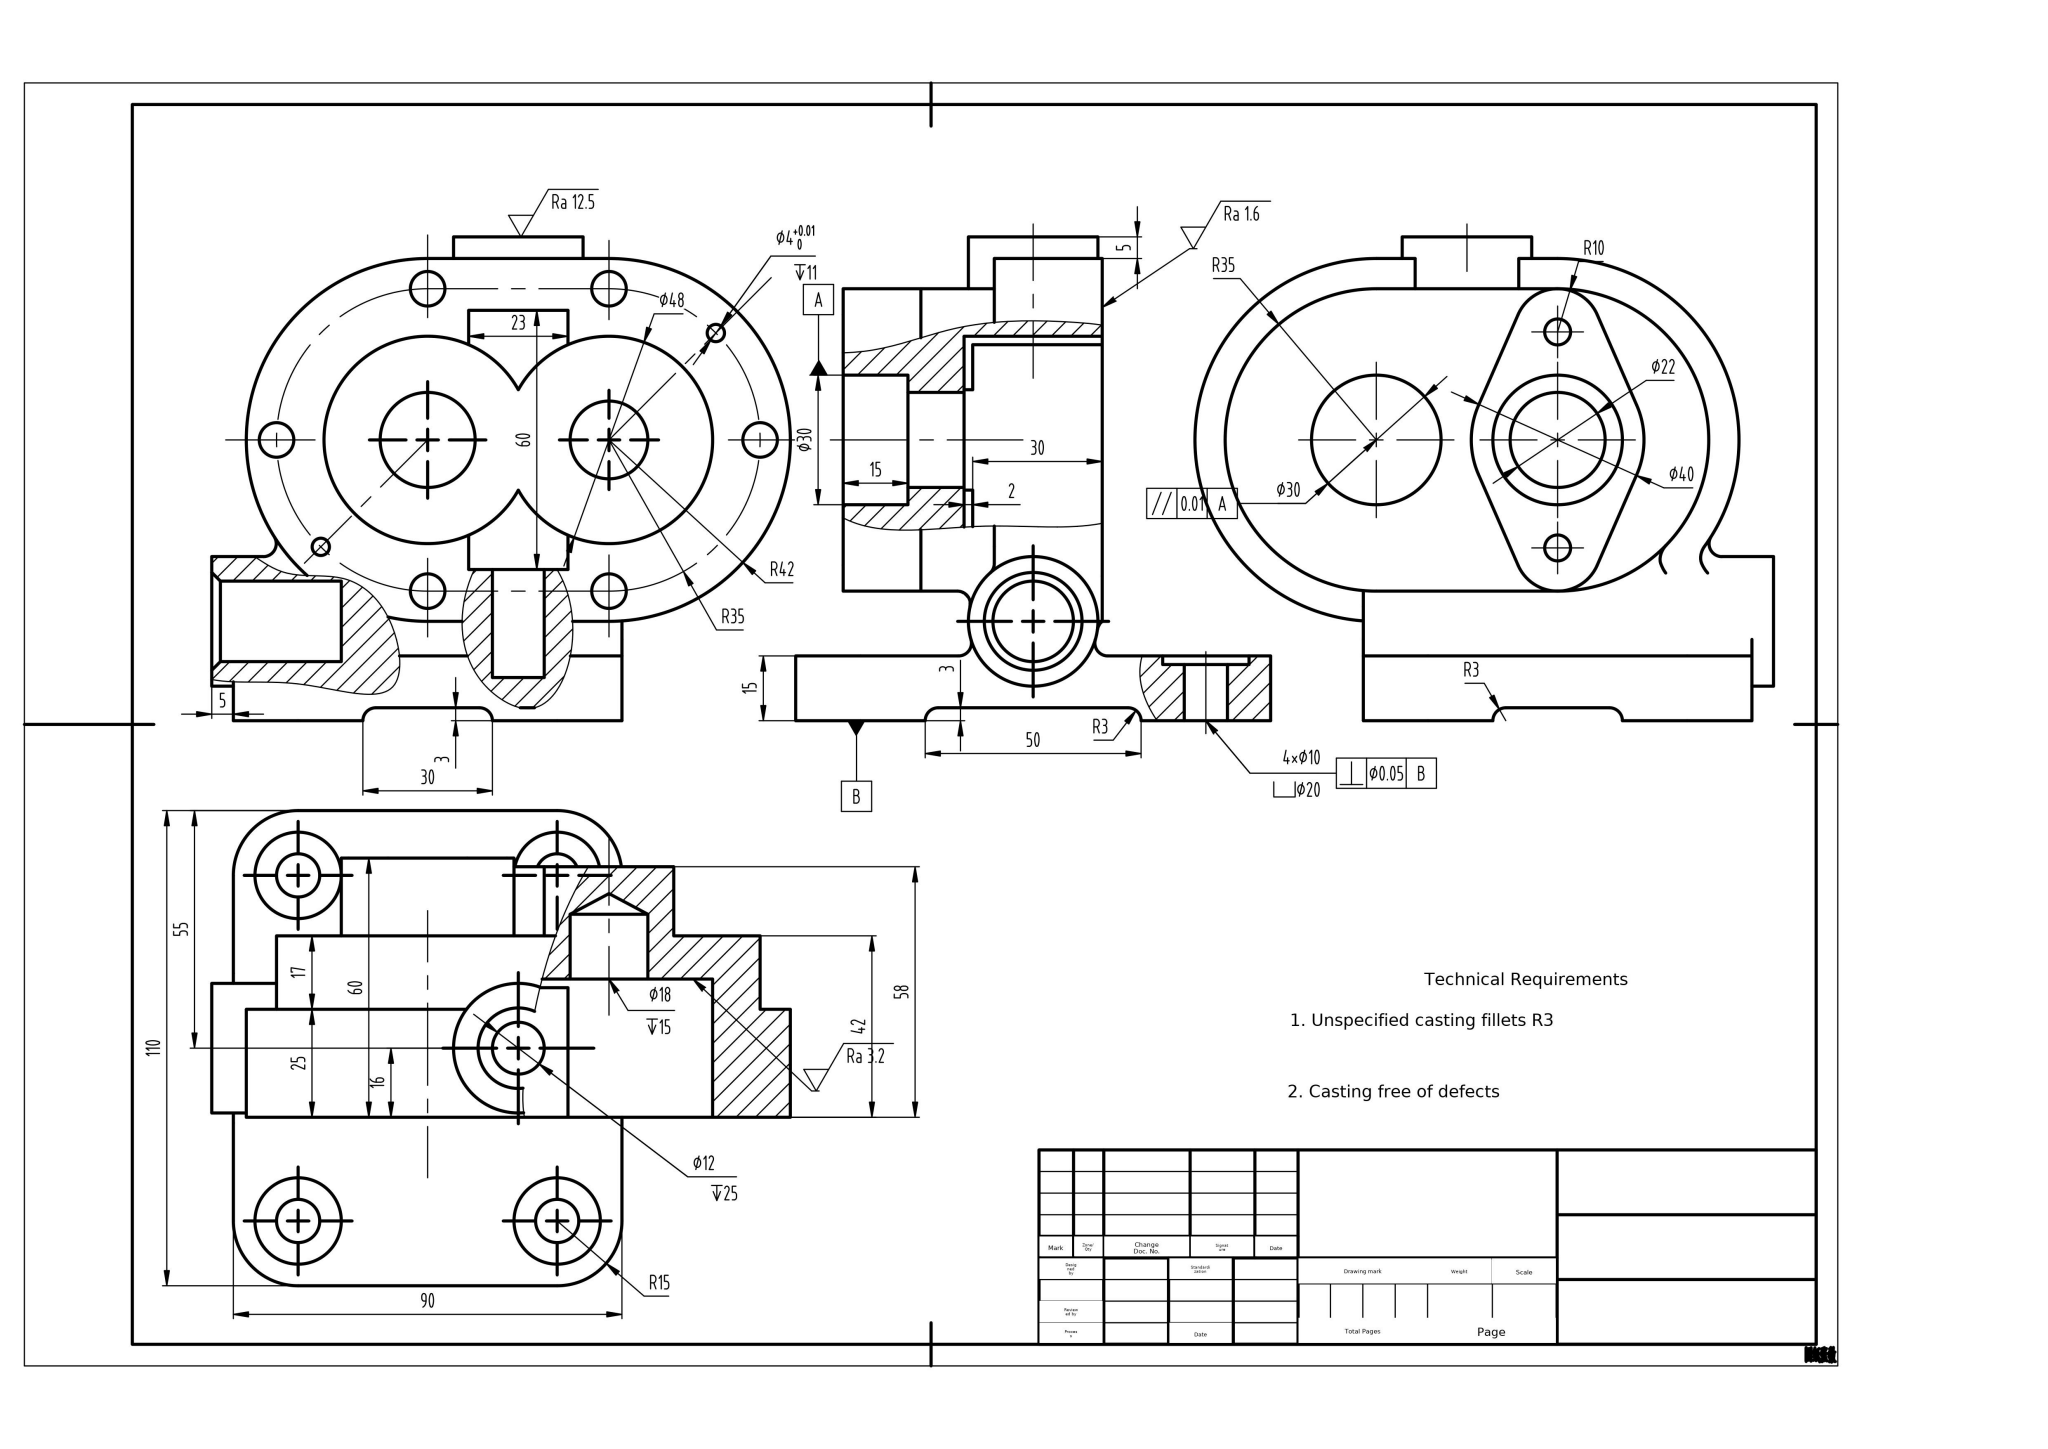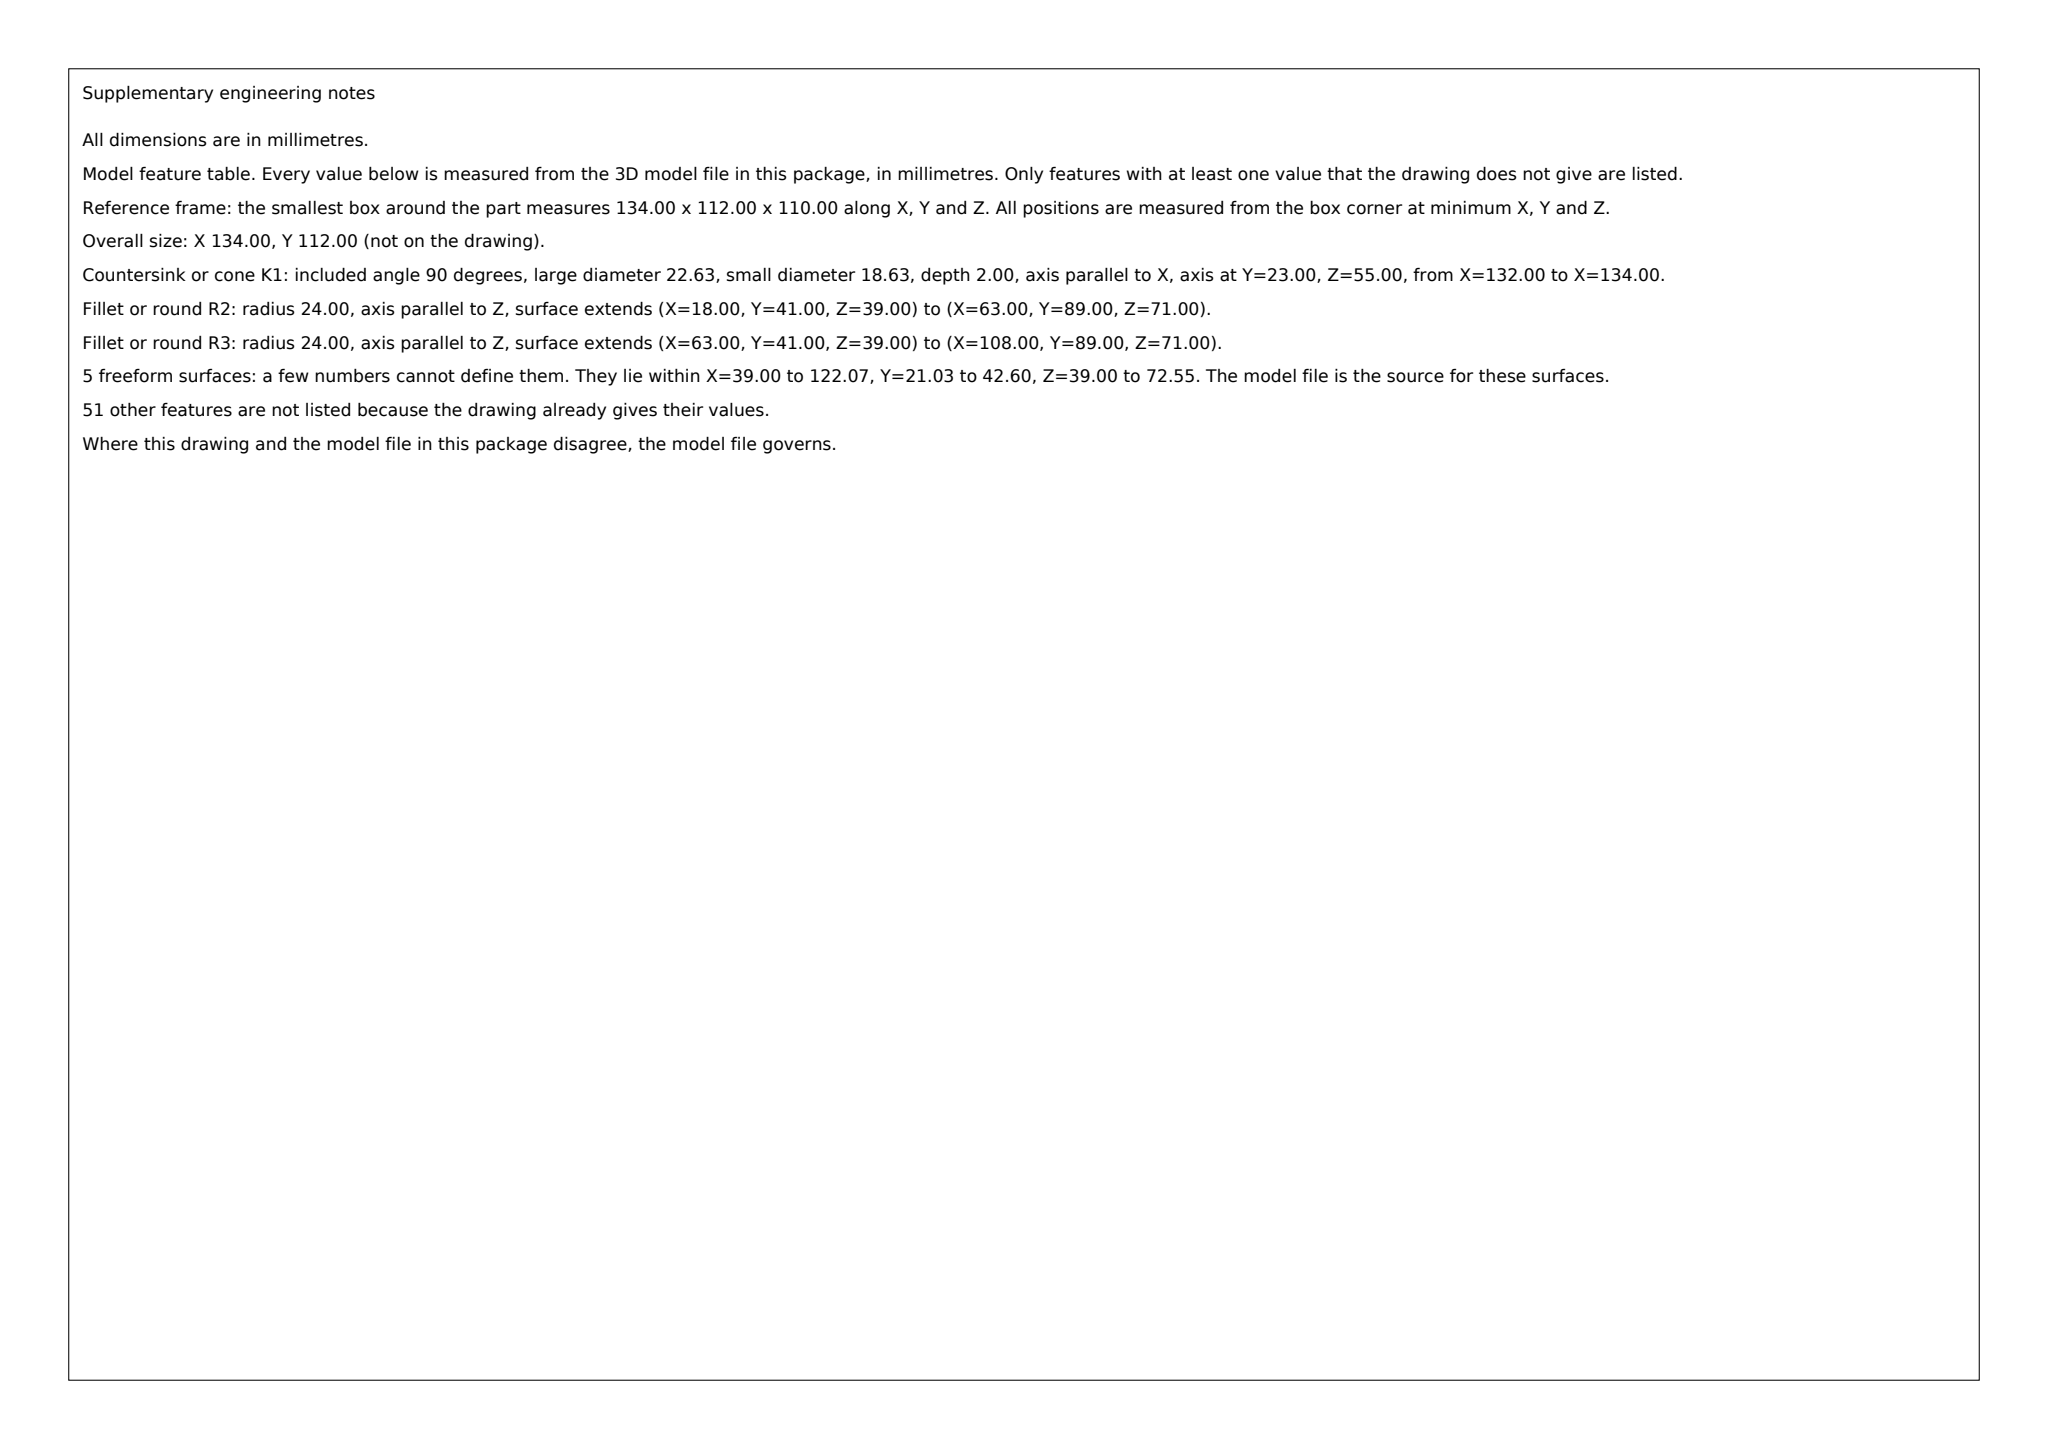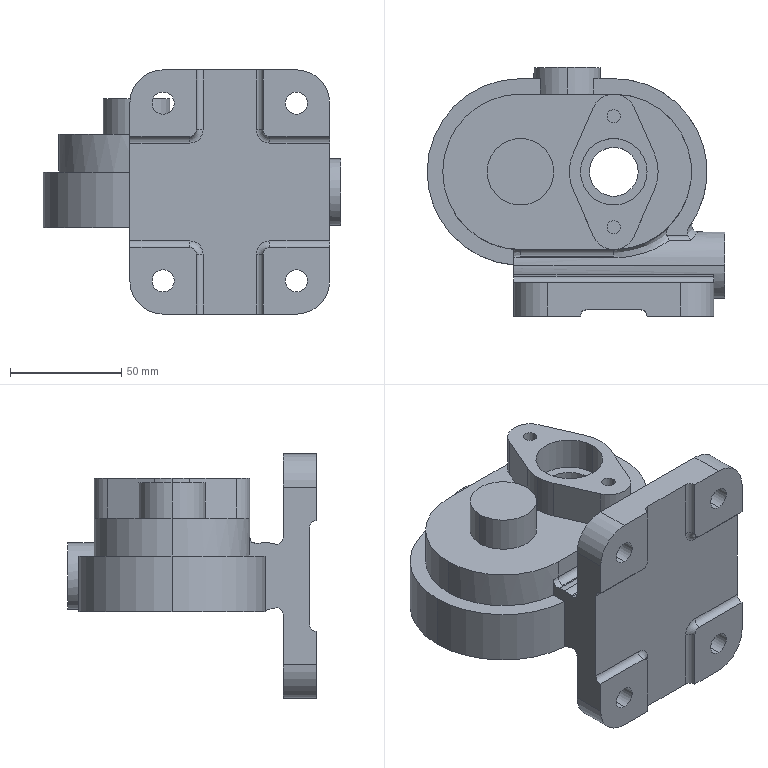Part | SolidWorks | mm | 1 solid | 152 faces | box 134 x 112 x 110 mm | volume 380839 mm3 | cylinder 87 | plane 54 | spline 5 | torus 4 | cone 2 | commonest cylinder face diameters 6 x19 8 x12 30 x12 20 x10 10 x8 18.632 x4 4 x4 48 x3